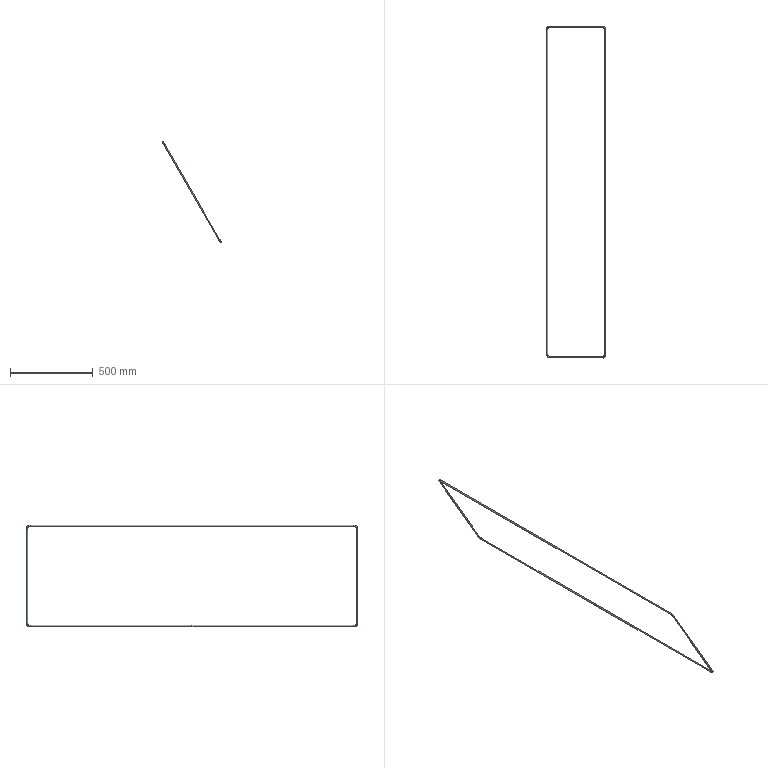Component | SolidWorks | FrontDoorAssembly-1_RubberPad-1 | 1 solid | 21 faces | box 358.69 x 2010 x 615.87 mm | volume 273869 mm3 | cylinder 10 | torus 8 | plane 3 | commonest cylinder face diameters 14.764 x10 | material Malleable Cast Iron
build123d program:
from build123d import *


with BuildPart() as part:
    # Sweep1: sweep along a path in Sketch2
    with BuildLine(Plane.XY) as sweep1_path:
        Line((0, 1), (0, 980))
        ThreePointArc((0, 980), (-5.858, 994.142), (-20, 1000))
        Line((-20, 1000), (-680, 1000))
        ThreePointArc((-680, 1000), (-694.142, 994.142), (-700, 980))
        Line((-700, 980), (-700, -980))
        ThreePointArc((-700, -980), (-694.142, -994.142), (-680, -1000))
        Line((-680, -1000), (-20, -1000))
        ThreePointArc((-20, -1000), (-5.858, -994.142), (0, -980))
        Line((0, -980), (0, 0))
    # Sketch3 → Sweep1 (sweep)
    with BuildSketch(Plane(origin=(0, 0, 0), x_dir=(1, 0, 0), z_dir=(0, 1, 0))):
        with BuildLine():
            Line((-5, -3.5), (5, -3.5))
            ThreePointArc((5, -3.5), (3.621, 0.7959), (0, 3.487))
            ThreePointArc((0, 3.487), (-3.621, 0.7959), (-5, -3.5))
        make_face()
    sweep(path=sweep1_path.line)


solid = part.part

# Placed as in the assembly
solid = solid.moved(Location((289.775, 925.17, 444.523), (0, 60, 0)))
STEP:
#1=COLOUR_RGB('',0.7922,0.8196,0.9333);
#2=FILL_AREA_STYLE_COLOUR('',#1);
#3=FILL_AREA_STYLE('',(#2));
#4=SURFACE_STYLE_FILL_AREA(#3);
#5=SURFACE_SIDE_STYLE('',(#4));
#6=SURFACE_STYLE_USAGE(.BOTH.,#5);
#7=PRESENTATION_STYLE_ASSIGNMENT((#6));
#8=CARTESIAN_POINT('',(11.626,75.007,17.399));
#9=VERTEX_POINT('',#8);
#10=CARTESIAN_POINT('',(11.29,75.007,17.432));
#11=VERTEX_POINT('',#10);
#12=CARTESIAN_POINT('',(11.481,75.007,17.651));
#13=DIRECTION('',(-0.,1.,0.));
#14=DIRECTION('',(0.866,0.,0.5));
#15=AXIS2_PLACEMENT_3D('',#12,#13,#14);
#16=CIRCLE('',#15,0.2906);
#17=EDGE_CURVE('',#9,#11,#16,.T.);
#18=ORIENTED_EDGE('',*,*,#17,.F.);
#19=CARTESIAN_POINT('',(11.626,36.463,17.399));
#20=VERTEX_POINT('',#19);
#21=CARTESIAN_POINT('',(11.626,75.007,17.399));
#22=DIRECTION('',(0.,-1.,-0.));
#23=VECTOR('',#22,39.37);
#24=LINE('',#21,#23);
#25=EDGE_CURVE('',#9,#20,#24,.T.);
#26=ORIENTED_EDGE('',*,*,#25,.T.);
#27=CARTESIAN_POINT('',(11.29,36.463,17.432));
#28=VERTEX_POINT('',#27);
#29=CARTESIAN_POINT('',(11.481,36.463,17.651));
#30=DIRECTION('',(-0.,1.,0.));
#31=DIRECTION('',(0.866,0.,0.5));
#32=AXIS2_PLACEMENT_3D('',#29,#30,#31);
#33=CIRCLE('',#32,0.2906);
#34=EDGE_CURVE('',#20,#28,#33,.T.);
#35=ORIENTED_EDGE('',*,*,#34,.T.);
#36=CARTESIAN_POINT('',(11.29,75.007,17.432));
#37=DIRECTION('',(0.,-1.,-0.));
#38=VECTOR('',#37,39.37);
#39=LINE('',#36,#38);
#40=EDGE_CURVE('',#11,#28,#39,.T.);
#41=ORIENTED_EDGE('',*,*,#40,.F.);
#42=EDGE_LOOP('',(#18,#26,#35,#41));
#43=FACE_OUTER_BOUND('',#42,.T.);
#44=CARTESIAN_POINT('',(11.481,75.007,17.651));
#45=DIRECTION('',(0.,-1.,-0.));
#46=DIRECTION('',(0.5,0.,-0.866));
#47=AXIS2_PLACEMENT_3D('',#44,#45,#46);
#48=CYLINDRICAL_SURFACE('',#47,0.2906);
#49=ADVANCED_FACE('',(#43),#48,.T.);
#50=CARTESIAN_POINT('',(11.429,75.007,17.74));
#51=VERTEX_POINT('',#50);
#52=CARTESIAN_POINT('',(11.575,75.007,17.489));
#53=DIRECTION('',(-0.,1.,0.));
#54=DIRECTION('',(-0.866,0.,-0.5));
#55=AXIS2_PLACEMENT_3D('',#52,#53,#54);
#56=CIRCLE('',#55,0.2906);
#57=EDGE_CURVE('',#11,#51,#56,.T.);
#58=ORIENTED_EDGE('',*,*,#57,.F.);
#59=ORIENTED_EDGE('',*,*,#40,.T.);
#60=CARTESIAN_POINT('',(11.429,36.463,17.74));
#61=VERTEX_POINT('',#60);
#62=CARTESIAN_POINT('',(11.575,36.463,17.489));
#63=DIRECTION('',(-0.,1.,0.));
#64=DIRECTION('',(-0.866,0.,-0.5));
#65=AXIS2_PLACEMENT_3D('',#62,#63,#64);
#66=CIRCLE('',#65,0.2906);
#67=EDGE_CURVE('',#28,#61,#66,.T.);
#68=ORIENTED_EDGE('',*,*,#67,.T.);
#69=CARTESIAN_POINT('',(11.429,75.007,17.74));
#70=DIRECTION('',(0.,-1.,-0.));
#71=VECTOR('',#70,39.37);
#72=LINE('',#69,#71);
#73=EDGE_CURVE('',#51,#61,#72,.T.);
#74=ORIENTED_EDGE('',*,*,#73,.F.);
#75=EDGE_LOOP('',(#58,#59,#68,#74));
#76=FACE_OUTER_BOUND('',#75,.T.);
#77=CARTESIAN_POINT('',(11.575,75.007,17.489));
#78=DIRECTION('',(0.,-1.,-0.));
#79=DIRECTION('',(0.5,0.,-0.866));
#80=AXIS2_PLACEMENT_3D('',#77,#78,#79);
#81=CYLINDRICAL_SURFACE('',#80,0.2906);
#82=ADVANCED_FACE('',(#76),#81,.T.);
#83=CARTESIAN_POINT('',(11.134,75.991,18.252));
#84=VERTEX_POINT('',#83);
#85=CARTESIAN_POINT('',(10.896,75.794,18.114));
#86=VERTEX_POINT('',#85);
#87=CARTESIAN_POINT('',(11.134,75.7,18.252));
#88=DIRECTION('',(-0.5,-0.,0.866));
#89=DIRECTION('',(0.866,0.,0.5));
#90=AXIS2_PLACEMENT_3D('',#87,#88,#89);
#91=CIRCLE('',#90,0.2906);
#92=EDGE_CURVE('',#84,#86,#91,.T.);
#93=ORIENTED_EDGE('',*,*,#92,.F.);
#94=CARTESIAN_POINT('',(11.134,75.007,18.252));
#95=DIRECTION('',(-0.866,-0.,-0.5));
#96=DIRECTION('',(-0.5,-0.,0.866));
#97=AXIS2_PLACEMENT_3D('',#94,#95,#96);
#98=CIRCLE('',#97,0.9843);
#99=EDGE_CURVE('',#84,#9,#98,.T.);
#100=ORIENTED_EDGE('',*,*,#99,.T.);
#101=ORIENTED_EDGE('',*,*,#17,.T.);
#102=CARTESIAN_POINT('',(10.896,75.007,18.114));
#103=DIRECTION('',(-0.866,-0.,-0.5));
#104=DIRECTION('',(-0.5,-0.,0.866));
#105=AXIS2_PLACEMENT_3D('',#102,#103,#104);
#106=CIRCLE('',#105,0.7874);
#107=EDGE_CURVE('',#86,#11,#106,.T.);
#108=ORIENTED_EDGE('',*,*,#107,.F.);
#109=EDGE_LOOP('',(#93,#100,#101,#108));
#110=FACE_OUTER_BOUND('',#109,.T.);
#111=CARTESIAN_POINT('',(11.134,75.007,18.252));
#112=DIRECTION('',(-0.866,-0.,-0.5));
#113=DIRECTION('',(-0.5,-0.,0.866));
#114=AXIS2_PLACEMENT_3D('',#111,#112,#113);
#115=TOROIDAL_SURFACE('',#114,0.6936,0.2906);
#116=ADVANCED_FACE('',(#110),#115,.T.);
#117=CARTESIAN_POINT('',(11.134,75.597,18.252));
#118=VERTEX_POINT('',#117);
#119=CARTESIAN_POINT('',(11.134,75.888,18.252));
#120=DIRECTION('',(-0.5,-0.,0.866));
#121=DIRECTION('',(-0.866,0.,-0.5));
#122=AXIS2_PLACEMENT_3D('',#119,#120,#121);
#123=CIRCLE('',#122,0.2906);
#124=EDGE_CURVE('',#86,#118,#123,.T.);
#125=ORIENTED_EDGE('',*,*,#124,.F.);
#126=ORIENTED_EDGE('',*,*,#107,.T.);
#127=ORIENTED_EDGE('',*,*,#57,.T.);
#128=CARTESIAN_POINT('',(11.134,75.007,18.252));
#129=DIRECTION('',(-0.866,-0.,-0.5));
#130=DIRECTION('',(-0.5,-0.,0.866));
#131=AXIS2_PLACEMENT_3D('',#128,#129,#130);
#132=CIRCLE('',#131,0.5906);
#133=EDGE_CURVE('',#118,#51,#132,.T.);
#134=ORIENTED_EDGE('',*,*,#133,.F.);
#135=EDGE_LOOP('',(#125,#126,#127,#134));
#136=FACE_OUTER_BOUND('',#135,.T.);
#137=CARTESIAN_POINT('',(11.134,75.007,18.252));
#138=DIRECTION('',(-0.866,-0.,-0.5));
#139=DIRECTION('',(-0.5,-0.,0.866));
#140=AXIS2_PLACEMENT_3D('',#137,#138,#139);
#141=TOROIDAL_SURFACE('',#140,0.8812,0.2906);
#142=ADVANCED_FACE('',(#136),#141,.T.);
#143=CARTESIAN_POINT('',(-1.858,75.991,40.755));
#144=VERTEX_POINT('',#143);
#145=CARTESIAN_POINT('',(-2.096,75.794,40.617));
#146=VERTEX_POINT('',#145);
#147=CARTESIAN_POINT('',(-1.858,75.7,40.755));
#148=DIRECTION('',(-0.5,-0.,0.866));
#149=DIRECTION('',(0.866,0.,0.5));
#150=AXIS2_PLACEMENT_3D('',#147,#148,#149);
#151=CIRCLE('',#150,0.2906);
#152=EDGE_CURVE('',#144,#146,#151,.T.);
#153=ORIENTED_EDGE('',*,*,#152,.F.);
#154=CARTESIAN_POINT('',(-1.858,75.991,40.755));
#155=DIRECTION('',(0.5,0.,-0.866));
#156=VECTOR('',#155,39.37);
#157=LINE('',#154,#156);
#158=EDGE_CURVE('',#144,#84,#157,.T.);
#159=ORIENTED_EDGE('',*,*,#158,.T.);
#160=ORIENTED_EDGE('',*,*,#92,.T.);
#161=CARTESIAN_POINT('',(-2.096,75.794,40.617));
#162=DIRECTION('',(0.5,0.,-0.866));
#163=VECTOR('',#162,39.37);
#164=LINE('',#161,#163);
#165=EDGE_CURVE('',#146,#86,#164,.T.);
#166=ORIENTED_EDGE('',*,*,#165,.F.);
#167=EDGE_LOOP('',(#153,#159,#160,#166));
#168=FACE_OUTER_BOUND('',#167,.T.);
#169=CARTESIAN_POINT('',(-1.858,75.7,40.755));
#170=DIRECTION('',(0.5,0.,-0.866));
#171=DIRECTION('',(-0.866,0.,-0.5));
#172=AXIS2_PLACEMENT_3D('',#169,#170,#171);
#173=CYLINDRICAL_SURFACE('',#172,0.2906);
#174=ADVANCED_FACE('',(#168),#173,.T.);
#175=CARTESIAN_POINT('',(-1.858,75.597,40.755));
#176=VERTEX_POINT('',#175);
#177=CARTESIAN_POINT('',(-1.858,75.888,40.755));
#178=DIRECTION('',(-0.5,-0.,0.866));
#179=DIRECTION('',(-0.866,0.,-0.5));
#180=AXIS2_PLACEMENT_3D('',#177,#178,#179);
#181=CIRCLE('',#180,0.2906);
#182=EDGE_CURVE('',#146,#176,#181,.T.);
#183=ORIENTED_EDGE('',*,*,#182,.F.);
#184=ORIENTED_EDGE('',*,*,#165,.T.);
#185=ORIENTED_EDGE('',*,*,#124,.T.);
#186=CARTESIAN_POINT('',(-1.858,75.597,40.755));
#187=DIRECTION('',(0.5,0.,-0.866));
#188=VECTOR('',#187,39.37);
#189=LINE('',#186,#188);
#190=EDGE_CURVE('',#176,#118,#189,.T.);
#191=ORIENTED_EDGE('',*,*,#190,.F.);
#192=EDGE_LOOP('',(#183,#184,#185,#191));
#193=FACE_OUTER_BOUND('',#192,.T.);
#194=CARTESIAN_POINT('',(-1.858,75.888,40.755));
#195=DIRECTION('',(0.5,0.,-0.866));
#196=DIRECTION('',(-0.866,0.,-0.5));
#197=AXIS2_PLACEMENT_3D('',#194,#195,#196);
#198=CYLINDRICAL_SURFACE('',#197,0.2906);
#199=ADVANCED_FACE('',(#193),#198,.T.);
#200=CARTESIAN_POINT('',(-2.35,75.007,41.607));
#201=VERTEX_POINT('',#200);
#202=CARTESIAN_POINT('',(-2.49,75.007,41.299));
#203=VERTEX_POINT('',#202);
#204=CARTESIAN_POINT('',(-2.205,75.007,41.355));
#205=DIRECTION('',(0.,-1.,-0.));
#206=DIRECTION('',(0.866,0.,0.5));
#207=AXIS2_PLACEMENT_3D('',#204,#205,#206);
#208=CIRCLE('',#207,0.2906);
#209=EDGE_CURVE('',#201,#203,#208,.T.);
#210=ORIENTED_EDGE('',*,*,#209,.F.);
#211=CARTESIAN_POINT('',(-1.858,75.007,40.755));
#212=DIRECTION('',(-0.866,-0.,-0.5));
#213=DIRECTION('',(-0.5,-0.,0.866));
#214=AXIS2_PLACEMENT_3D('',#211,#212,#213);
#215=CIRCLE('',#214,0.9843);
#216=EDGE_CURVE('',#201,#144,#215,.T.);
#217=ORIENTED_EDGE('',*,*,#216,.T.);
#218=ORIENTED_EDGE('',*,*,#152,.T.);
#219=CARTESIAN_POINT('',(-2.096,75.007,40.617));
#220=DIRECTION('',(-0.866,-0.,-0.5));
#221=DIRECTION('',(-0.5,-0.,0.866));
#222=AXIS2_PLACEMENT_3D('',#219,#220,#221);
#223=CIRCLE('',#222,0.7874);
#224=EDGE_CURVE('',#203,#146,#223,.T.);
#225=ORIENTED_EDGE('',*,*,#224,.F.);
#226=EDGE_LOOP('',(#210,#217,#218,#225));
#227=FACE_OUTER_BOUND('',#226,.T.);
#228=CARTESIAN_POINT('',(-1.858,75.007,40.755));
#229=DIRECTION('',(-0.866,-0.,-0.5));
#230=DIRECTION('',(-0.5,-0.,0.866));
#231=AXIS2_PLACEMENT_3D('',#228,#229,#230);
#232=TOROIDAL_SURFACE('',#231,0.6936,0.2906);
#233=ADVANCED_FACE('',(#227),#232,.T.);
#234=CARTESIAN_POINT('',(-2.153,75.007,41.266));
#235=VERTEX_POINT('',#234);
#236=CARTESIAN_POINT('',(-2.299,75.007,41.518));
#237=DIRECTION('',(0.,-1.,-0.));
#238=DIRECTION('',(-0.866,0.,-0.5));
#239=AXIS2_PLACEMENT_3D('',#236,#237,#238);
#240=CIRCLE('',#239,0.2906);
#241=EDGE_CURVE('',#203,#235,#240,.T.);
#242=ORIENTED_EDGE('',*,*,#241,.F.);
#243=ORIENTED_EDGE('',*,*,#224,.T.);
#244=ORIENTED_EDGE('',*,*,#182,.T.);
#245=CARTESIAN_POINT('',(-1.858,75.007,40.755));
#246=DIRECTION('',(-0.866,-0.,-0.5));
#247=DIRECTION('',(-0.5,-0.,0.866));
#248=AXIS2_PLACEMENT_3D('',#245,#246,#247);
#249=CIRCLE('',#248,0.5906);
#250=EDGE_CURVE('',#235,#176,#249,.T.);
#251=ORIENTED_EDGE('',*,*,#250,.F.);
#252=EDGE_LOOP('',(#242,#243,#244,#251));
#253=FACE_OUTER_BOUND('',#252,.T.);
#254=CARTESIAN_POINT('',(-1.858,75.007,40.755));
#255=DIRECTION('',(-0.866,-0.,-0.5));
#256=DIRECTION('',(-0.5,-0.,0.866));
#257=AXIS2_PLACEMENT_3D('',#254,#255,#256);
#258=TOROIDAL_SURFACE('',#257,0.8812,0.2906);
#259=ADVANCED_FACE('',(#253),#258,.T.);
#260=CARTESIAN_POINT('',(-2.35,-2.159,41.607));
#261=VERTEX_POINT('',#260);
#262=CARTESIAN_POINT('',(-2.49,-2.159,41.299));
#263=VERTEX_POINT('',#262);
#264=CARTESIAN_POINT('',(-2.205,-2.159,41.355));
#265=DIRECTION('',(0.,-1.,-0.));
#266=DIRECTION('',(0.866,0.,0.5));
#267=AXIS2_PLACEMENT_3D('',#264,#265,#266);
#268=CIRCLE('',#267,0.2906);
#269=EDGE_CURVE('',#261,#263,#268,.T.);
#270=ORIENTED_EDGE('',*,*,#269,.F.);
#271=CARTESIAN_POINT('',(-2.35,-2.159,41.607));
#272=DIRECTION('',(-0.,1.,0.));
#273=VECTOR('',#272,39.37);
#274=LINE('',#271,#273);
#275=EDGE_CURVE('',#261,#201,#274,.T.);
#276=ORIENTED_EDGE('',*,*,#275,.T.);
#277=ORIENTED_EDGE('',*,*,#209,.T.);
#278=CARTESIAN_POINT('',(-2.49,-2.159,41.299));
#279=DIRECTION('',(-0.,1.,0.));
#280=VECTOR('',#279,39.37);
#281=LINE('',#278,#280);
#282=EDGE_CURVE('',#263,#203,#281,.T.);
#283=ORIENTED_EDGE('',*,*,#282,.F.);
#284=EDGE_LOOP('',(#270,#276,#277,#283));
#285=FACE_OUTER_BOUND('',#284,.T.);
#286=CARTESIAN_POINT('',(-2.205,-2.159,41.355));
#287=DIRECTION('',(-0.,1.,0.));
#288=DIRECTION('',(-0.5,-0.,0.866));
#289=AXIS2_PLACEMENT_3D('',#286,#287,#288);
#290=CYLINDRICAL_SURFACE('',#289,0.2906);
#291=ADVANCED_FACE('',(#285),#290,.T.);
#292=CARTESIAN_POINT('',(-2.153,-2.159,41.266));
#293=VERTEX_POINT('',#292);
#294=CARTESIAN_POINT('',(-2.299,-2.159,41.518));
#295=DIRECTION('',(0.,-1.,-0.));
#296=DIRECTION('',(-0.866,-0.,-0.5));
#297=AXIS2_PLACEMENT_3D('',#294,#295,#296);
#298=CIRCLE('',#297,0.2906);
#299=EDGE_CURVE('',#263,#293,#298,.T.);
#300=ORIENTED_EDGE('',*,*,#299,.F.);
#301=ORIENTED_EDGE('',*,*,#282,.T.);
#302=ORIENTED_EDGE('',*,*,#241,.T.);
#303=CARTESIAN_POINT('',(-2.153,-2.159,41.266));
#304=DIRECTION('',(-0.,1.,0.));
#305=VECTOR('',#304,39.37);
#306=LINE('',#303,#305);
#307=EDGE_CURVE('',#293,#235,#306,.T.);
#308=ORIENTED_EDGE('',*,*,#307,.F.);
#309=EDGE_LOOP('',(#300,#301,#302,#308));
#310=FACE_OUTER_BOUND('',#309,.T.);
#311=CARTESIAN_POINT('',(-2.299,-2.159,41.518));
#312=DIRECTION('',(-0.,1.,0.));
#313=DIRECTION('',(-0.5,-0.,0.866));
#314=AXIS2_PLACEMENT_3D('',#311,#312,#313);
#315=CYLINDRICAL_SURFACE('',#314,0.2906);
#316=ADVANCED_FACE('',(#310),#315,.T.);
#317=CARTESIAN_POINT('',(-1.858,-3.143,40.755));
#318=VERTEX_POINT('',#317);
#319=CARTESIAN_POINT('',(-2.096,-2.946,40.617));
#320=VERTEX_POINT('',#319);
#321=CARTESIAN_POINT('',(-1.858,-2.852,40.755));
#322=DIRECTION('',(0.5,0.,-0.866));
#323=DIRECTION('',(0.866,0.,0.5));
#324=AXIS2_PLACEMENT_3D('',#321,#322,#323);
#325=CIRCLE('',#324,0.2906);
#326=EDGE_CURVE('',#318,#320,#325,.T.);
#327=ORIENTED_EDGE('',*,*,#326,.F.);
#328=CARTESIAN_POINT('',(-1.858,-2.159,40.755));
#329=DIRECTION('',(-0.866,-0.,-0.5));
#330=DIRECTION('',(-0.5,-0.,0.866));
#331=AXIS2_PLACEMENT_3D('',#328,#329,#330);
#332=CIRCLE('',#331,0.9843);
#333=EDGE_CURVE('',#318,#261,#332,.T.);
#334=ORIENTED_EDGE('',*,*,#333,.T.);
#335=ORIENTED_EDGE('',*,*,#269,.T.);
#336=CARTESIAN_POINT('',(-2.096,-2.159,40.617));
#337=DIRECTION('',(-0.866,-0.,-0.5));
#338=DIRECTION('',(-0.5,-0.,0.866));
#339=AXIS2_PLACEMENT_3D('',#336,#337,#338);
#340=CIRCLE('',#339,0.7874);
#341=EDGE_CURVE('',#320,#263,#340,.T.);
#342=ORIENTED_EDGE('',*,*,#341,.F.);
#343=EDGE_LOOP('',(#327,#334,#335,#342));
#344=FACE_OUTER_BOUND('',#343,.T.);
#345=CARTESIAN_POINT('',(-1.858,-2.159,40.755));
#346=DIRECTION('',(-0.866,-0.,-0.5));
#347=DIRECTION('',(-0.5,-0.,0.866));
#348=AXIS2_PLACEMENT_3D('',#345,#346,#347);
#349=TOROIDAL_SURFACE('',#348,0.6936,0.2906);
#350=ADVANCED_FACE('',(#344),#349,.T.);
#351=CARTESIAN_POINT('',(-1.858,-2.749,40.755));
#352=VERTEX_POINT('',#351);
#353=CARTESIAN_POINT('',(-1.858,-3.04,40.755));
#354=DIRECTION('',(0.5,0.,-0.866));
#355=DIRECTION('',(-0.866,-0.,-0.5));
#356=AXIS2_PLACEMENT_3D('',#353,#354,#355);
#357=CIRCLE('',#356,0.2906);
#358=EDGE_CURVE('',#320,#352,#357,.T.);
#359=ORIENTED_EDGE('',*,*,#358,.F.);
#360=ORIENTED_EDGE('',*,*,#341,.T.);
#361=ORIENTED_EDGE('',*,*,#299,.T.);
#362=CARTESIAN_POINT('',(-1.858,-2.159,40.755));
#363=DIRECTION('',(-0.866,-0.,-0.5));
#364=DIRECTION('',(-0.5,-0.,0.866));
#365=AXIS2_PLACEMENT_3D('',#362,#363,#364);
#366=CIRCLE('',#365,0.5906);
#367=EDGE_CURVE('',#352,#293,#366,.T.);
#368=ORIENTED_EDGE('',*,*,#367,.F.);
#369=EDGE_LOOP('',(#359,#360,#361,#368));
#370=FACE_OUTER_BOUND('',#369,.T.);
#371=CARTESIAN_POINT('',(-1.858,-2.159,40.755));
#372=DIRECTION('',(-0.866,-0.,-0.5));
#373=DIRECTION('',(-0.5,-0.,0.866));
#374=AXIS2_PLACEMENT_3D('',#371,#372,#373);
#375=TOROIDAL_SURFACE('',#374,0.8812,0.2906);
#376=ADVANCED_FACE('',(#370),#375,.T.);
#377=CARTESIAN_POINT('',(11.134,-3.143,18.252));
#378=VERTEX_POINT('',#377);
#379=CARTESIAN_POINT('',(10.896,-2.946,18.114));
#380=VERTEX_POINT('',#379);
#381=CARTESIAN_POINT('',(11.134,-2.852,18.252));
#382=DIRECTION('',(0.5,0.,-0.866));
#383=DIRECTION('',(0.866,0.,0.5));
#384=AXIS2_PLACEMENT_3D('',#381,#382,#383);
#385=CIRCLE('',#384,0.2906);
#386=EDGE_CURVE('',#378,#380,#385,.T.);
#387=ORIENTED_EDGE('',*,*,#386,.F.);
#388=CARTESIAN_POINT('',(11.134,-3.143,18.252));
#389=DIRECTION('',(-0.5,-0.,0.866));
#390=VECTOR('',#389,39.37);
#391=LINE('',#388,#390);
#392=EDGE_CURVE('',#378,#318,#391,.T.);
#393=ORIENTED_EDGE('',*,*,#392,.T.);
#394=ORIENTED_EDGE('',*,*,#326,.T.);
#395=CARTESIAN_POINT('',(10.896,-2.946,18.114));
#396=DIRECTION('',(-0.5,-0.,0.866));
#397=VECTOR('',#396,39.37);
#398=LINE('',#395,#397);
#399=EDGE_CURVE('',#380,#320,#398,.T.);
#400=ORIENTED_EDGE('',*,*,#399,.F.);
#401=EDGE_LOOP('',(#387,#393,#394,#400));
#402=FACE_OUTER_BOUND('',#401,.T.);
#403=CARTESIAN_POINT('',(11.134,-2.852,18.252));
#404=DIRECTION('',(-0.5,-0.,0.866));
#405=DIRECTION('',(0.866,0.,0.5));
#406=AXIS2_PLACEMENT_3D('',#403,#404,#405);
#407=CYLINDRICAL_SURFACE('',#406,0.2906);
#408=ADVANCED_FACE('',(#402),#407,.T.);
#409=CARTESIAN_POINT('',(11.134,-2.749,18.252));
#410=VERTEX_POINT('',#409);
#411=CARTESIAN_POINT('',(11.134,-3.04,18.252));
#412=DIRECTION('',(0.5,0.,-0.866));
#413=DIRECTION('',(-0.866,-0.,-0.5));
#414=AXIS2_PLACEMENT_3D('',#411,#412,#413);
#415=CIRCLE('',#414,0.2906);
#416=EDGE_CURVE('',#380,#410,#415,.T.);
#417=ORIENTED_EDGE('',*,*,#416,.F.);
#418=ORIENTED_EDGE('',*,*,#399,.T.);
#419=ORIENTED_EDGE('',*,*,#358,.T.);
#420=CARTESIAN_POINT('',(11.134,-2.749,18.252));
#421=DIRECTION('',(-0.5,-0.,0.866));
#422=VECTOR('',#421,39.37);
#423=LINE('',#420,#422);
#424=EDGE_CURVE('',#410,#352,#423,.T.);
#425=ORIENTED_EDGE('',*,*,#424,.F.);
#426=EDGE_LOOP('',(#417,#418,#419,#425));
#427=FACE_OUTER_BOUND('',#426,.T.);
#428=CARTESIAN_POINT('',(11.134,-3.04,18.252));
#429=DIRECTION('',(-0.5,-0.,0.866));
#430=DIRECTION('',(0.866,0.,0.5));
#431=AXIS2_PLACEMENT_3D('',#428,#429,#430);
#432=CYLINDRICAL_SURFACE('',#431,0.2906);
#433=ADVANCED_FACE('',(#427),#432,.T.);
#434=CARTESIAN_POINT('',(11.626,-2.159,17.399));
#435=VERTEX_POINT('',#434);
#436=CARTESIAN_POINT('',(11.29,-2.159,17.432));
#437=VERTEX_POINT('',#436);
#438=CARTESIAN_POINT('',(11.481,-2.159,17.651));
#439=DIRECTION('',(-0.,1.,0.));
#440=DIRECTION('',(0.866,0.,0.5));
#441=AXIS2_PLACEMENT_3D('',#438,#439,#440);
#442=CIRCLE('',#441,0.2906);
#443=EDGE_CURVE('',#435,#437,#442,.T.);
#444=ORIENTED_EDGE('',*,*,#443,.F.);
#445=CARTESIAN_POINT('',(11.134,-2.159,18.252));
#446=DIRECTION('',(-0.866,-0.,-0.5));
#447=DIRECTION('',(-0.5,-0.,0.866));
#448=AXIS2_PLACEMENT_3D('',#445,#446,#447);
#449=CIRCLE('',#448,0.9843);
#450=EDGE_CURVE('',#435,#378,#449,.T.);
#451=ORIENTED_EDGE('',*,*,#450,.T.);
#452=ORIENTED_EDGE('',*,*,#386,.T.);
#453=CARTESIAN_POINT('',(10.896,-2.159,18.114));
#454=DIRECTION('',(-0.866,-0.,-0.5));
#455=DIRECTION('',(-0.5,-0.,0.866));
#456=AXIS2_PLACEMENT_3D('',#453,#454,#455);
#457=CIRCLE('',#456,0.7874);
#458=EDGE_CURVE('',#437,#380,#457,.T.);
#459=ORIENTED_EDGE('',*,*,#458,.F.);
#460=EDGE_LOOP('',(#444,#451,#452,#459));
#461=FACE_OUTER_BOUND('',#460,.T.);
#462=CARTESIAN_POINT('',(11.134,-2.159,18.252));
#463=DIRECTION('',(-0.866,-0.,-0.5));
#464=DIRECTION('',(-0.5,-0.,0.866));
#465=AXIS2_PLACEMENT_3D('',#462,#463,#464);
#466=TOROIDAL_SURFACE('',#465,0.6936,0.2906);
#467=ADVANCED_FACE('',(#461),#466,.T.);
#468=CARTESIAN_POINT('',(11.429,-2.159,17.74));
#469=VERTEX_POINT('',#468);
#470=CARTESIAN_POINT('',(11.575,-2.159,17.489));
#471=DIRECTION('',(-0.,1.,0.));
#472=DIRECTION('',(-0.866,-0.,-0.5));
#473=AXIS2_PLACEMENT_3D('',#470,#471,#472);
#474=CIRCLE('',#473,0.2906);
#475=EDGE_CURVE('',#437,#469,#474,.T.);
#476=ORIENTED_EDGE('',*,*,#475,.F.);
#477=ORIENTED_EDGE('',*,*,#458,.T.);
#478=ORIENTED_EDGE('',*,*,#416,.T.);
#479=CARTESIAN_POINT('',(11.134,-2.159,18.252));
#480=DIRECTION('',(-0.866,-0.,-0.5));
#481=DIRECTION('',(-0.5,-0.,0.866));
#482=AXIS2_PLACEMENT_3D('',#479,#480,#481);
#483=CIRCLE('',#482,0.5906);
#484=EDGE_CURVE('',#469,#410,#483,.T.);
#485=ORIENTED_EDGE('',*,*,#484,.F.);
#486=EDGE_LOOP('',(#476,#477,#478,#485));
#487=FACE_OUTER_BOUND('',#486,.T.);
#488=CARTESIAN_POINT('',(11.134,-2.159,18.252));
#489=DIRECTION('',(-0.866,-0.,-0.5));
#490=DIRECTION('',(-0.5,-0.,0.866));
#491=AXIS2_PLACEMENT_3D('',#488,#489,#490);
#492=TOROIDAL_SURFACE('',#491,0.8812,0.2906);
#493=ADVANCED_FACE('',(#487),#492,.T.);
#494=CARTESIAN_POINT('',(11.29,36.424,17.432));
#495=VERTEX_POINT('',#494);
#496=CARTESIAN_POINT('',(11.429,36.424,17.74));
#497=VERTEX_POINT('',#496);
#498=CARTESIAN_POINT('',(11.575,36.424,17.489));
#499=DIRECTION('',(-0.,1.,0.));
#500=DIRECTION('',(-0.866,0.,-0.5));
#501=AXIS2_PLACEMENT_3D('',#498,#499,#500);
#502=CIRCLE('',#501,0.2906);
#503=EDGE_CURVE('',#495,#497,#502,.T.);
#504=ORIENTED_EDGE('',*,*,#503,.F.);
#505=CARTESIAN_POINT('',(11.29,-2.159,17.432));
#506=DIRECTION('',(-0.,1.,0.));
#507=VECTOR('',#506,39.37);
#508=LINE('',#505,#507);
#509=EDGE_CURVE('',#437,#495,#508,.T.);
#510=ORIENTED_EDGE('',*,*,#509,.F.);
#511=ORIENTED_EDGE('',*,*,#475,.T.);
#512=CARTESIAN_POINT('',(11.429,-2.159,17.74));
#513=DIRECTION('',(-0.,1.,0.));
#514=VECTOR('',#513,39.37);
#515=LINE('',#512,#514);
#516=EDGE_CURVE('',#469,#497,#515,.T.);
#517=ORIENTED_EDGE('',*,*,#516,.T.);
#518=EDGE_LOOP('',(#504,#510,#511,#517));
#519=FACE_OUTER_BOUND('',#518,.T.);
#520=CARTESIAN_POINT('',(11.575,-2.159,17.489));
#521=DIRECTION('',(-0.,1.,0.));
#522=DIRECTION('',(-0.5,-0.,0.866));
#523=AXIS2_PLACEMENT_3D('',#520,#521,#522);
#524=CYLINDRICAL_SURFACE('',#523,0.2906);
#525=ADVANCED_FACE('',(#519),#524,.T.);
#526=CARTESIAN_POINT('',(11.626,36.424,17.399));
#527=VERTEX_POINT('',#526);
#528=CARTESIAN_POINT('',(11.481,36.424,17.651));
#529=DIRECTION('',(-0.,1.,0.));
#530=DIRECTION('',(0.866,0.,0.5));
#531=AXIS2_PLACEMENT_3D('',#528,#529,#530);
#532=CIRCLE('',#531,0.2906);
#533=EDGE_CURVE('',#527,#495,#532,.T.);
#534=ORIENTED_EDGE('',*,*,#533,.F.);
#535=CARTESIAN_POINT('',(11.626,-2.159,17.399));
#536=DIRECTION('',(-0.,1.,0.));
#537=VECTOR('',#536,39.37);
#538=LINE('',#535,#537);
#539=EDGE_CURVE('',#435,#527,#538,.T.);
#540=ORIENTED_EDGE('',*,*,#539,.F.);
#541=ORIENTED_EDGE('',*,*,#443,.T.);
#542=ORIENTED_EDGE('',*,*,#509,.T.);
#543=EDGE_LOOP('',(#534,#540,#541,#542));
#544=FACE_OUTER_BOUND('',#543,.T.);
#545=CARTESIAN_POINT('',(11.481,-2.159,17.651));
#546=DIRECTION('',(-0.,1.,0.));
#547=DIRECTION('',(-0.5,-0.,0.866));
#548=AXIS2_PLACEMENT_3D('',#545,#546,#547);
#549=CYLINDRICAL_SURFACE('',#548,0.2906);
#550=ADVANCED_FACE('',(#544),#549,.T.);
#551=CARTESIAN_POINT('',(11.429,36.424,17.74));
#552=DIRECTION('',(0.5,0.,-0.866));
#553=VECTOR('',#552,39.37);
#554=LINE('',#551,#553);
#555=EDGE_CURVE('',#497,#527,#554,.T.);
#556=ORIENTED_EDGE('',*,*,#555,.F.);
#557=ORIENTED_EDGE('',*,*,#516,.F.);
#558=ORIENTED_EDGE('',*,*,#484,.T.);
#559=ORIENTED_EDGE('',*,*,#424,.T.);
#560=ORIENTED_EDGE('',*,*,#367,.T.);
#561=ORIENTED_EDGE('',*,*,#307,.T.);
#562=ORIENTED_EDGE('',*,*,#250,.T.);
#563=ORIENTED_EDGE('',*,*,#190,.T.);
#564=ORIENTED_EDGE('',*,*,#133,.T.);
#565=ORIENTED_EDGE('',*,*,#73,.T.);
#566=CARTESIAN_POINT('',(11.429,36.463,17.74));
#567=DIRECTION('',(0.5,0.,-0.866));
#568=VECTOR('',#567,39.37);
#569=LINE('',#566,#568);
#570=EDGE_CURVE('',#61,#20,#569,.T.);
#571=ORIENTED_EDGE('',*,*,#570,.T.);
#572=ORIENTED_EDGE('',*,*,#25,.F.);
#573=ORIENTED_EDGE('',*,*,#99,.F.);
#574=ORIENTED_EDGE('',*,*,#158,.F.);
#575=ORIENTED_EDGE('',*,*,#216,.F.);
#576=ORIENTED_EDGE('',*,*,#275,.F.);
#577=ORIENTED_EDGE('',*,*,#333,.F.);
#578=ORIENTED_EDGE('',*,*,#392,.F.);
#579=ORIENTED_EDGE('',*,*,#450,.F.);
#580=ORIENTED_EDGE('',*,*,#539,.T.);
#581=EDGE_LOOP('',(#556,#557,#558,#559,#560,#561,#562,#563,#564,#565,#571,#572,#573,#574,#575,#576,#577,#578,#579,#580));
#582=FACE_OUTER_BOUND('',#581,.T.);
#583=CARTESIAN_POINT('',(11.429,-2.159,17.74));
#584=DIRECTION('',(0.866,0.,0.5));
#585=DIRECTION('',(0.5,0.,-0.866));
#586=AXIS2_PLACEMENT_3D('',#583,#584,#585);
#587=PLANE('',#586);
#588=ADVANCED_FACE('',(#582),#587,.T.);
#589=ORIENTED_EDGE('',*,*,#67,.F.);
#590=ORIENTED_EDGE('',*,*,#34,.F.);
#591=ORIENTED_EDGE('',*,*,#570,.F.);
#592=EDGE_LOOP('',(#589,#590,#591));
#593=FACE_OUTER_BOUND('',#592,.T.);
#594=CARTESIAN_POINT('',(11.575,36.463,17.489));
#595=DIRECTION('',(0.,-1.,-0.));
#596=DIRECTION('',(-0.866,-0.,-0.5));
#597=AXIS2_PLACEMENT_3D('',#594,#595,#596);
#598=PLANE('',#597);
#599=ADVANCED_FACE('',(#593),#598,.T.);
#600=ORIENTED_EDGE('',*,*,#503,.T.);
#601=ORIENTED_EDGE('',*,*,#555,.T.);
#602=ORIENTED_EDGE('',*,*,#533,.T.);
#603=EDGE_LOOP('',(#600,#601,#602));
#604=FACE_OUTER_BOUND('',#603,.T.);
#605=CARTESIAN_POINT('',(11.575,36.424,17.489));
#606=DIRECTION('',(0.,-1.,-0.));
#607=DIRECTION('',(-0.866,-0.,-0.5));
#608=AXIS2_PLACEMENT_3D('',#605,#606,#607);
#609=PLANE('',#608);
#610=ADVANCED_FACE('',(#604),#609,.F.);
#611=CLOSED_SHELL('',(#49,#82,#116,#142,#174,#199,#233,#259,#291,#316,#350,#376,#408,#433,#467,#493,#525,#550,#588,#599,#610));
#612=MANIFOLD_SOLID_BREP('',#611);
#613=STYLED_ITEM('',(#7),#612);
#614=(LENGTH_UNIT()NAMED_UNIT(*)SI_UNIT($,.METRE.));
#615=LENGTH_MEASURE_WITH_UNIT(LENGTH_MEASURE(0.0254),#614);
#616=DIMENSIONAL_EXPONENTS(1.,0.,0.,0.,0.,0.,0.);
#617=(CONVERSION_BASED_UNIT('',#615)LENGTH_UNIT()NAMED_UNIT(#616));
#618=UNCERTAINTY_MEASURE_WITH_UNIT(LENGTH_MEASURE(0.00001),#617,'','');
#619=(NAMED_UNIT(*)PLANE_ANGLE_UNIT()SI_UNIT($,.RADIAN.));
#620=(NAMED_UNIT(*)SI_UNIT($,.STERADIAN.)SOLID_ANGLE_UNIT());
#621=(GEOMETRIC_REPRESENTATION_CONTEXT(3)GLOBAL_UNCERTAINTY_ASSIGNED_CONTEXT((#618))GLOBAL_UNIT_ASSIGNED_CONTEXT((#617,#619,#620))REPRESENTATION_CONTEXT('',''));
#622=MECHANICAL_DESIGN_GEOMETRIC_PRESENTATION_REPRESENTATION('',(#613),#621);
#623=CARTESIAN_POINT('',(0.,0.,0.));
#624=DIRECTION('',(0.,0.,1.));
#625=DIRECTION('',(1.,0.,0.));
#626=AXIS2_PLACEMENT_3D('',#623,#624,#625);
#627=(LENGTH_UNIT()NAMED_UNIT(*)SI_UNIT($,.METRE.));
#628=LENGTH_MEASURE_WITH_UNIT(LENGTH_MEASURE(0.0254),#627);
#629=DIMENSIONAL_EXPONENTS(1.,0.,0.,0.,0.,0.,0.);
#630=(CONVERSION_BASED_UNIT('',#628)LENGTH_UNIT()NAMED_UNIT(#629));
#631=UNCERTAINTY_MEASURE_WITH_UNIT(LENGTH_MEASURE(0.00001),#630,'','');
#632=(NAMED_UNIT(*)PLANE_ANGLE_UNIT()SI_UNIT($,.RADIAN.));
#633=(NAMED_UNIT(*)SI_UNIT($,.STERADIAN.)SOLID_ANGLE_UNIT());
#634=(GEOMETRIC_REPRESENTATION_CONTEXT(3)GLOBAL_UNCERTAINTY_ASSIGNED_CONTEXT((#631))GLOBAL_UNIT_ASSIGNED_CONTEXT((#630,#632,#633))REPRESENTATION_CONTEXT('',''));
#635=ADVANCED_BREP_SHAPE_REPRESENTATION('',(#612,#626),#634);
#636=PRESENTATION_LAYER_ASSIGNMENT('','',(#613));